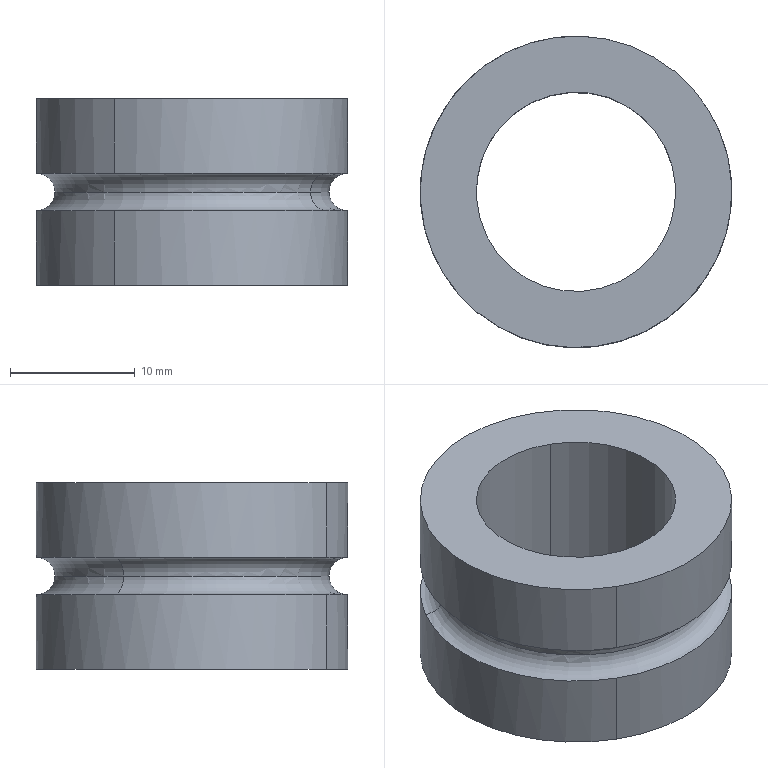Component | SolidWorks | SpindleFixtureAssemblyLeft-1_KLHFH016_16CopperSleeve-2 | 1 solid | 12 faces | box 25 x 25 x 15 mm | volume 4084 mm3 | cylinder 6 | torus 4 | plane 2 | commonest cylinder face diameters 25 x4 16 x2 | material Brass
build123d program:
from build123d import *

# Parameters (mm, degrees)
SKETCH1_R           = 12.5
SKETCH1_R_2         = 8
BOSS_EXTRUDE1_DEPTH = 7.5
SKETCH2_R           = 1.5


with BuildPart() as part:
    # Sketch1 → Boss-Extrude1 (new, symmetric)
    with BuildSketch(Plane.XY):
        Circle(SKETCH1_R)
        Circle(SKETCH1_R_2, mode=Mode.SUBTRACT)
    extrude(amount=BOSS_EXTRUDE1_DEPTH, both=True)

    # Sketch2 → Cut-Revolve1 (revolve, cut)
    with BuildSketch(Plane(origin=(0, 0, 0), x_dir=(0, 0, -1), z_dir=(1, 0, 0)), mode=Mode.PRIVATE) as cut_revolve1_sk:
        with Locations((0, 12.5)):
            Circle(SKETCH2_R)
    revolve(cut_revolve1_sk.sketch.rotate(Axis((0, 0, 0), (0, 0, -1)), 180), axis=Axis((0, 0, 0), (0, 0, -1)), mode=Mode.SUBTRACT)


solid = part.part

# Placed as in the assembly
solid = solid.moved(Location((-25, -43.301, -218.5), (0, 0, 0)))
STEP:
#1=CARTESIAN_POINT('',(-1.41,-1.459,-8.661));
#2=VERTEX_POINT('',#1);
#3=CARTESIAN_POINT('',(-1.359,-1.488,-8.602));
#4=VERTEX_POINT('',#3);
#5=CARTESIAN_POINT('',(-1.41,-1.459,-8.602));
#6=DIRECTION('',(-0.5,-0.866,0.));
#7=DIRECTION('',(0.866,-0.5,0.));
#8=AXIS2_PLACEMENT_3D('',#5,#6,#7);
#9=CIRCLE('',#8,0.05906);
#10=EDGE_CURVE('',#2,#4,#9,.T.);
#11=ORIENTED_EDGE('',*,*,#10,.T.);
#12=CARTESIAN_POINT('',(-0.6092,-1.921,-8.602));
#13=VERTEX_POINT('',#12);
#14=CARTESIAN_POINT('',(-0.9843,-1.705,-8.602));
#15=DIRECTION('',(0.,-0.,-1.));
#16=DIRECTION('',(-1.,0.,0.));
#17=AXIS2_PLACEMENT_3D('',#14,#15,#16);
#18=CIRCLE('',#17,0.4331);
#19=EDGE_CURVE('',#4,#13,#18,.T.);
#20=ORIENTED_EDGE('',*,*,#19,.T.);
#21=CARTESIAN_POINT('',(-0.5581,-1.951,-8.661));
#22=VERTEX_POINT('',#21);
#23=CARTESIAN_POINT('',(-0.5581,-1.951,-8.602));
#24=DIRECTION('',(0.5,0.866,-0.));
#25=DIRECTION('',(-0.866,0.5,0.));
#26=AXIS2_PLACEMENT_3D('',#23,#24,#25);
#27=CIRCLE('',#26,0.05906);
#28=EDGE_CURVE('',#22,#13,#27,.T.);
#29=ORIENTED_EDGE('',*,*,#28,.F.);
#30=CARTESIAN_POINT('',(-0.7382,-1.279,-8.661));
#31=VERTEX_POINT('',#30);
#32=CARTESIAN_POINT('',(-0.9843,-1.705,-8.661));
#33=DIRECTION('',(-0.,0.,1.));
#34=DIRECTION('',(0.866,-0.5,0.));
#35=AXIS2_PLACEMENT_3D('',#32,#33,#34);
#36=CIRCLE('',#35,0.4921);
#37=EDGE_CURVE('',#22,#31,#36,.T.);
#38=ORIENTED_EDGE('',*,*,#37,.T.);
#39=CARTESIAN_POINT('',(-0.9843,-1.705,-8.661));
#40=DIRECTION('',(-0.,0.,1.));
#41=DIRECTION('',(0.866,-0.5,0.));
#42=AXIS2_PLACEMENT_3D('',#39,#40,#41);
#43=CIRCLE('',#42,0.4921);
#44=EDGE_CURVE('',#31,#2,#43,.T.);
#45=ORIENTED_EDGE('',*,*,#44,.T.);
#46=EDGE_LOOP('',(#11,#20,#29,#38,#45));
#47=FACE_OUTER_BOUND('',#46,.T.);
#48=CARTESIAN_POINT('',(-0.9843,-1.705,-8.602));
#49=DIRECTION('',(0.,-0.,-1.));
#50=DIRECTION('',(-0.866,0.5,-0.));
#51=AXIS2_PLACEMENT_3D('',#48,#49,#50);
#52=TOROIDAL_SURFACE('',#51,0.4921,0.05906);
#53=ADVANCED_FACE('',(#47),#52,.F.);
#54=ORIENTED_EDGE('',*,*,#28,.T.);
#55=CARTESIAN_POINT('',(-0.9843,-1.705,-8.602));
#56=DIRECTION('',(0.,-0.,-1.));
#57=DIRECTION('',(-1.,0.,0.));
#58=AXIS2_PLACEMENT_3D('',#55,#56,#57);
#59=CIRCLE('',#58,0.4331);
#60=EDGE_CURVE('',#13,#4,#59,.T.);
#61=ORIENTED_EDGE('',*,*,#60,.T.);
#62=ORIENTED_EDGE('',*,*,#10,.F.);
#63=CARTESIAN_POINT('',(-1.23,-2.131,-8.661));
#64=VERTEX_POINT('',#63);
#65=CARTESIAN_POINT('',(-0.9843,-1.705,-8.661));
#66=DIRECTION('',(-0.,0.,1.));
#67=DIRECTION('',(0.866,-0.5,0.));
#68=AXIS2_PLACEMENT_3D('',#65,#66,#67);
#69=CIRCLE('',#68,0.4921);
#70=EDGE_CURVE('',#2,#64,#69,.T.);
#71=ORIENTED_EDGE('',*,*,#70,.T.);
#72=CARTESIAN_POINT('',(-0.9843,-1.705,-8.661));
#73=DIRECTION('',(-0.,0.,1.));
#74=DIRECTION('',(0.866,-0.5,0.));
#75=AXIS2_PLACEMENT_3D('',#72,#73,#74);
#76=CIRCLE('',#75,0.4921);
#77=EDGE_CURVE('',#64,#22,#76,.T.);
#78=ORIENTED_EDGE('',*,*,#77,.T.);
#79=EDGE_LOOP('',(#54,#61,#62,#71,#78));
#80=FACE_OUTER_BOUND('',#79,.T.);
#81=CARTESIAN_POINT('',(-0.9843,-1.705,-8.602));
#82=DIRECTION('',(0.,-0.,-1.));
#83=DIRECTION('',(-0.866,0.5,-0.));
#84=AXIS2_PLACEMENT_3D('',#81,#82,#83);
#85=TOROIDAL_SURFACE('',#84,0.4921,0.05906);
#86=ADVANCED_FACE('',(#80),#85,.F.);
#87=ORIENTED_EDGE('',*,*,#60,.F.);
#88=CARTESIAN_POINT('',(-0.5581,-1.951,-8.543));
#89=VERTEX_POINT('',#88);
#90=CARTESIAN_POINT('',(-0.5581,-1.951,-8.602));
#91=DIRECTION('',(0.5,0.866,-0.));
#92=DIRECTION('',(-0.866,0.5,0.));
#93=AXIS2_PLACEMENT_3D('',#90,#91,#92);
#94=CIRCLE('',#93,0.05906);
#95=EDGE_CURVE('',#13,#89,#94,.T.);
#96=ORIENTED_EDGE('',*,*,#95,.T.);
#97=CARTESIAN_POINT('',(-1.23,-2.131,-8.543));
#98=VERTEX_POINT('',#97);
#99=CARTESIAN_POINT('',(-0.9843,-1.705,-8.543));
#100=DIRECTION('',(0.,-0.,-1.));
#101=DIRECTION('',(-0.866,0.5,0.));
#102=AXIS2_PLACEMENT_3D('',#99,#100,#101);
#103=CIRCLE('',#102,0.4921);
#104=EDGE_CURVE('',#89,#98,#103,.T.);
#105=ORIENTED_EDGE('',*,*,#104,.T.);
#106=CARTESIAN_POINT('',(-1.41,-1.459,-8.543));
#107=VERTEX_POINT('',#106);
#108=CARTESIAN_POINT('',(-0.9843,-1.705,-8.543));
#109=DIRECTION('',(0.,-0.,-1.));
#110=DIRECTION('',(-0.866,0.5,0.));
#111=AXIS2_PLACEMENT_3D('',#108,#109,#110);
#112=CIRCLE('',#111,0.4921);
#113=EDGE_CURVE('',#98,#107,#112,.T.);
#114=ORIENTED_EDGE('',*,*,#113,.T.);
#115=CARTESIAN_POINT('',(-1.41,-1.459,-8.602));
#116=DIRECTION('',(-0.5,-0.866,0.));
#117=DIRECTION('',(0.866,-0.5,0.));
#118=AXIS2_PLACEMENT_3D('',#115,#116,#117);
#119=CIRCLE('',#118,0.05906);
#120=EDGE_CURVE('',#4,#107,#119,.T.);
#121=ORIENTED_EDGE('',*,*,#120,.F.);
#122=EDGE_LOOP('',(#87,#96,#105,#114,#121));
#123=FACE_OUTER_BOUND('',#122,.T.);
#124=CARTESIAN_POINT('',(-0.9843,-1.705,-8.602));
#125=DIRECTION('',(0.,-0.,-1.));
#126=DIRECTION('',(-0.866,0.5,-0.));
#127=AXIS2_PLACEMENT_3D('',#124,#125,#126);
#128=TOROIDAL_SURFACE('',#127,0.4921,0.05906);
#129=ADVANCED_FACE('',(#123),#128,.F.);
#130=CARTESIAN_POINT('',(-1.142,-1.978,-8.898));
#131=VERTEX_POINT('',#130);
#132=CARTESIAN_POINT('',(-0.8268,-1.432,-8.898));
#133=VERTEX_POINT('',#132);
#134=CARTESIAN_POINT('',(-0.9843,-1.705,-8.898));
#135=DIRECTION('',(0.,0.,-1.));
#136=DIRECTION('',(0.5,0.866,0.));
#137=AXIS2_PLACEMENT_3D('',#134,#135,#136);
#138=CIRCLE('',#137,0.315);
#139=EDGE_CURVE('',#131,#133,#138,.T.);
#140=ORIENTED_EDGE('',*,*,#139,.T.);
#141=CARTESIAN_POINT('',(-0.8268,-1.432,-8.307));
#142=VERTEX_POINT('',#141);
#143=CARTESIAN_POINT('',(-0.8268,-1.432,-8.898));
#144=DIRECTION('',(0.,0.,1.));
#145=VECTOR('',#144,39.37);
#146=LINE('',#143,#145);
#147=EDGE_CURVE('',#133,#142,#146,.T.);
#148=ORIENTED_EDGE('',*,*,#147,.T.);
#149=CARTESIAN_POINT('',(-1.142,-1.978,-8.307));
#150=VERTEX_POINT('',#149);
#151=CARTESIAN_POINT('',(-0.9843,-1.705,-8.307));
#152=DIRECTION('',(0.,0.,-1.));
#153=DIRECTION('',(0.5,0.866,0.));
#154=AXIS2_PLACEMENT_3D('',#151,#152,#153);
#155=CIRCLE('',#154,0.315);
#156=EDGE_CURVE('',#150,#142,#155,.T.);
#157=ORIENTED_EDGE('',*,*,#156,.F.);
#158=CARTESIAN_POINT('',(-1.142,-1.978,-8.898));
#159=DIRECTION('',(0.,0.,1.));
#160=VECTOR('',#159,39.37);
#161=LINE('',#158,#160);
#162=EDGE_CURVE('',#131,#150,#161,.T.);
#163=ORIENTED_EDGE('',*,*,#162,.F.);
#164=EDGE_LOOP('',(#140,#148,#157,#163));
#165=FACE_OUTER_BOUND('',#164,.T.);
#166=CARTESIAN_POINT('',(-0.9843,-1.705,-8.898));
#167=DIRECTION('',(0.,0.,1.));
#168=DIRECTION('',(-0.5,-0.866,0.));
#169=AXIS2_PLACEMENT_3D('',#166,#167,#168);
#170=CYLINDRICAL_SURFACE('',#169,0.315);
#171=ADVANCED_FACE('',(#165),#170,.F.);
#172=CARTESIAN_POINT('',(-0.7382,-1.279,-8.543));
#173=VERTEX_POINT('',#172);
#174=CARTESIAN_POINT('',(-0.9843,-1.705,-8.543));
#175=DIRECTION('',(0.,-0.,-1.));
#176=DIRECTION('',(-0.866,0.5,0.));
#177=AXIS2_PLACEMENT_3D('',#174,#175,#176);
#178=CIRCLE('',#177,0.4921);
#179=EDGE_CURVE('',#173,#89,#178,.T.);
#180=ORIENTED_EDGE('',*,*,#179,.F.);
#181=CARTESIAN_POINT('',(-0.7382,-1.279,-8.307));
#182=VERTEX_POINT('',#181);
#183=CARTESIAN_POINT('',(-0.7382,-1.279,-8.898));
#184=DIRECTION('',(0.,0.,1.));
#185=VECTOR('',#184,39.37);
#186=LINE('',#183,#185);
#187=EDGE_CURVE('',#173,#182,#186,.T.);
#188=ORIENTED_EDGE('',*,*,#187,.T.);
#189=CARTESIAN_POINT('',(-1.23,-2.131,-8.307));
#190=VERTEX_POINT('',#189);
#191=CARTESIAN_POINT('',(-0.9843,-1.705,-8.307));
#192=DIRECTION('',(0.,0.,-1.));
#193=DIRECTION('',(0.5,0.866,0.));
#194=AXIS2_PLACEMENT_3D('',#191,#192,#193);
#195=CIRCLE('',#194,0.4921);
#196=EDGE_CURVE('',#182,#190,#195,.T.);
#197=ORIENTED_EDGE('',*,*,#196,.T.);
#198=CARTESIAN_POINT('',(-1.23,-2.131,-8.898));
#199=DIRECTION('',(0.,0.,1.));
#200=VECTOR('',#199,39.37);
#201=LINE('',#198,#200);
#202=EDGE_CURVE('',#98,#190,#201,.T.);
#203=ORIENTED_EDGE('',*,*,#202,.F.);
#204=ORIENTED_EDGE('',*,*,#104,.F.);
#205=EDGE_LOOP('',(#180,#188,#197,#203,#204));
#206=FACE_OUTER_BOUND('',#205,.T.);
#207=CARTESIAN_POINT('',(-0.9843,-1.705,-8.898));
#208=DIRECTION('',(0.,0.,1.));
#209=DIRECTION('',(-0.5,-0.866,0.));
#210=AXIS2_PLACEMENT_3D('',#207,#208,#209);
#211=CYLINDRICAL_SURFACE('',#210,0.4921);
#212=ADVANCED_FACE('',(#206),#211,.T.);
#213=CARTESIAN_POINT('',(-0.7382,-1.279,-8.898));
#214=VERTEX_POINT('',#213);
#215=CARTESIAN_POINT('',(-1.23,-2.131,-8.898));
#216=VERTEX_POINT('',#215);
#217=CARTESIAN_POINT('',(-0.9843,-1.705,-8.898));
#218=DIRECTION('',(0.,0.,-1.));
#219=DIRECTION('',(0.5,0.866,0.));
#220=AXIS2_PLACEMENT_3D('',#217,#218,#219);
#221=CIRCLE('',#220,0.4921);
#222=EDGE_CURVE('',#214,#216,#221,.T.);
#223=ORIENTED_EDGE('',*,*,#222,.F.);
#224=CARTESIAN_POINT('',(-0.7382,-1.279,-8.898));
#225=DIRECTION('',(0.,0.,1.));
#226=VECTOR('',#225,39.37);
#227=LINE('',#224,#226);
#228=EDGE_CURVE('',#214,#31,#227,.T.);
#229=ORIENTED_EDGE('',*,*,#228,.T.);
#230=ORIENTED_EDGE('',*,*,#37,.F.);
#231=ORIENTED_EDGE('',*,*,#77,.F.);
#232=CARTESIAN_POINT('',(-1.23,-2.131,-8.898));
#233=DIRECTION('',(0.,0.,1.));
#234=VECTOR('',#233,39.37);
#235=LINE('',#232,#234);
#236=EDGE_CURVE('',#216,#64,#235,.T.);
#237=ORIENTED_EDGE('',*,*,#236,.F.);
#238=EDGE_LOOP('',(#223,#229,#230,#231,#237));
#239=FACE_OUTER_BOUND('',#238,.T.);
#240=CARTESIAN_POINT('',(-0.9843,-1.705,-8.898));
#241=DIRECTION('',(0.,0.,1.));
#242=DIRECTION('',(-0.5,-0.866,0.));
#243=AXIS2_PLACEMENT_3D('',#240,#241,#242);
#244=CYLINDRICAL_SURFACE('',#243,0.4921);
#245=ADVANCED_FACE('',(#239),#244,.T.);
#246=ORIENTED_EDGE('',*,*,#228,.F.);
#247=CARTESIAN_POINT('',(-0.9843,-1.705,-8.898));
#248=DIRECTION('',(0.,0.,-1.));
#249=DIRECTION('',(0.5,0.866,0.));
#250=AXIS2_PLACEMENT_3D('',#247,#248,#249);
#251=CIRCLE('',#250,0.4921);
#252=EDGE_CURVE('',#216,#214,#251,.T.);
#253=ORIENTED_EDGE('',*,*,#252,.F.);
#254=ORIENTED_EDGE('',*,*,#236,.T.);
#255=ORIENTED_EDGE('',*,*,#70,.F.);
#256=ORIENTED_EDGE('',*,*,#44,.F.);
#257=EDGE_LOOP('',(#246,#253,#254,#255,#256));
#258=FACE_OUTER_BOUND('',#257,.T.);
#259=CARTESIAN_POINT('',(-0.9843,-1.705,-8.898));
#260=DIRECTION('',(0.,0.,1.));
#261=DIRECTION('',(-0.5,-0.866,0.));
#262=AXIS2_PLACEMENT_3D('',#259,#260,#261);
#263=CYLINDRICAL_SURFACE('',#262,0.4921);
#264=ADVANCED_FACE('',(#258),#263,.T.);
#265=ORIENTED_EDGE('',*,*,#187,.F.);
#266=CARTESIAN_POINT('',(-0.9843,-1.705,-8.543));
#267=DIRECTION('',(0.,-0.,-1.));
#268=DIRECTION('',(-0.866,0.5,0.));
#269=AXIS2_PLACEMENT_3D('',#266,#267,#268);
#270=CIRCLE('',#269,0.4921);
#271=EDGE_CURVE('',#107,#173,#270,.T.);
#272=ORIENTED_EDGE('',*,*,#271,.F.);
#273=ORIENTED_EDGE('',*,*,#113,.F.);
#274=ORIENTED_EDGE('',*,*,#202,.T.);
#275=CARTESIAN_POINT('',(-0.9843,-1.705,-8.307));
#276=DIRECTION('',(0.,0.,-1.));
#277=DIRECTION('',(0.5,0.866,0.));
#278=AXIS2_PLACEMENT_3D('',#275,#276,#277);
#279=CIRCLE('',#278,0.4921);
#280=EDGE_CURVE('',#190,#182,#279,.T.);
#281=ORIENTED_EDGE('',*,*,#280,.T.);
#282=EDGE_LOOP('',(#265,#272,#273,#274,#281));
#283=FACE_OUTER_BOUND('',#282,.T.);
#284=CARTESIAN_POINT('',(-0.9843,-1.705,-8.898));
#285=DIRECTION('',(0.,0.,1.));
#286=DIRECTION('',(-0.5,-0.866,0.));
#287=AXIS2_PLACEMENT_3D('',#284,#285,#286);
#288=CYLINDRICAL_SURFACE('',#287,0.4921);
#289=ADVANCED_FACE('',(#283),#288,.T.);
#290=ORIENTED_EDGE('',*,*,#252,.T.);
#291=ORIENTED_EDGE('',*,*,#222,.T.);
#292=EDGE_LOOP('',(#290,#291));
#293=FACE_OUTER_BOUND('',#292,.T.);
#294=ORIENTED_EDGE('',*,*,#139,.F.);
#295=CARTESIAN_POINT('',(-0.9843,-1.705,-8.898));
#296=DIRECTION('',(0.,0.,-1.));
#297=DIRECTION('',(0.5,0.866,0.));
#298=AXIS2_PLACEMENT_3D('',#295,#296,#297);
#299=CIRCLE('',#298,0.315);
#300=EDGE_CURVE('',#133,#131,#299,.T.);
#301=ORIENTED_EDGE('',*,*,#300,.F.);
#302=EDGE_LOOP('',(#294,#301));
#303=FACE_BOUND('',#302,.T.);
#304=CARTESIAN_POINT('',(-0.9843,-1.705,-8.898));
#305=DIRECTION('',(0.,0.,-1.));
#306=DIRECTION('',(0.5,0.866,0.));
#307=AXIS2_PLACEMENT_3D('',#304,#305,#306);
#308=PLANE('',#307);
#309=ADVANCED_FACE('',(#293,#303),#308,.T.);
#310=ORIENTED_EDGE('',*,*,#280,.F.);
#311=ORIENTED_EDGE('',*,*,#196,.F.);
#312=EDGE_LOOP('',(#310,#311));
#313=FACE_OUTER_BOUND('',#312,.T.);
#314=ORIENTED_EDGE('',*,*,#156,.T.);
#315=CARTESIAN_POINT('',(-0.9843,-1.705,-8.307));
#316=DIRECTION('',(0.,0.,-1.));
#317=DIRECTION('',(0.5,0.866,0.));
#318=AXIS2_PLACEMENT_3D('',#315,#316,#317);
#319=CIRCLE('',#318,0.315);
#320=EDGE_CURVE('',#142,#150,#319,.T.);
#321=ORIENTED_EDGE('',*,*,#320,.T.);
#322=EDGE_LOOP('',(#314,#321));
#323=FACE_BOUND('',#322,.T.);
#324=CARTESIAN_POINT('',(-0.9843,-1.705,-8.307));
#325=DIRECTION('',(0.,0.,-1.));
#326=DIRECTION('',(0.5,0.866,0.));
#327=AXIS2_PLACEMENT_3D('',#324,#325,#326);
#328=PLANE('',#327);
#329=ADVANCED_FACE('',(#313,#323),#328,.F.);
#330=ORIENTED_EDGE('',*,*,#147,.F.);
#331=ORIENTED_EDGE('',*,*,#300,.T.);
#332=ORIENTED_EDGE('',*,*,#162,.T.);
#333=ORIENTED_EDGE('',*,*,#320,.F.);
#334=EDGE_LOOP('',(#330,#331,#332,#333));
#335=FACE_OUTER_BOUND('',#334,.T.);
#336=CARTESIAN_POINT('',(-0.9843,-1.705,-8.898));
#337=DIRECTION('',(0.,0.,1.));
#338=DIRECTION('',(-0.5,-0.866,0.));
#339=AXIS2_PLACEMENT_3D('',#336,#337,#338);
#340=CYLINDRICAL_SURFACE('',#339,0.315);
#341=ADVANCED_FACE('',(#335),#340,.F.);
#342=ORIENTED_EDGE('',*,*,#19,.F.);
#343=ORIENTED_EDGE('',*,*,#120,.T.);
#344=ORIENTED_EDGE('',*,*,#271,.T.);
#345=ORIENTED_EDGE('',*,*,#179,.T.);
#346=ORIENTED_EDGE('',*,*,#95,.F.);
#347=EDGE_LOOP('',(#342,#343,#344,#345,#346));
#348=FACE_OUTER_BOUND('',#347,.T.);
#349=CARTESIAN_POINT('',(-0.9843,-1.705,-8.602));
#350=DIRECTION('',(0.,-0.,-1.));
#351=DIRECTION('',(-0.866,0.5,-0.));
#352=AXIS2_PLACEMENT_3D('',#349,#350,#351);
#353=TOROIDAL_SURFACE('',#352,0.4921,0.05906);
#354=ADVANCED_FACE('',(#348),#353,.F.);
#355=CLOSED_SHELL('',(#53,#86,#129,#171,#212,#245,#264,#289,#309,#329,#341,#354));
#356=MANIFOLD_SOLID_BREP('',#355);
#357=CARTESIAN_POINT('',(0.,0.,0.));
#358=DIRECTION('',(0.,0.,1.));
#359=DIRECTION('',(1.,0.,0.));
#360=AXIS2_PLACEMENT_3D('',#357,#358,#359);
#361=(LENGTH_UNIT()NAMED_UNIT(*)SI_UNIT($,.METRE.));
#362=LENGTH_MEASURE_WITH_UNIT(LENGTH_MEASURE(0.0254),#361);
#363=DIMENSIONAL_EXPONENTS(1.,0.,0.,0.,0.,0.,0.);
#364=(CONVERSION_BASED_UNIT('',#362)LENGTH_UNIT()NAMED_UNIT(#363));
#365=UNCERTAINTY_MEASURE_WITH_UNIT(LENGTH_MEASURE(0.00001),#364,'','');
#366=(NAMED_UNIT(*)PLANE_ANGLE_UNIT()SI_UNIT($,.RADIAN.));
#367=(NAMED_UNIT(*)SI_UNIT($,.STERADIAN.)SOLID_ANGLE_UNIT());
#368=(GEOMETRIC_REPRESENTATION_CONTEXT(3)GLOBAL_UNCERTAINTY_ASSIGNED_CONTEXT((#365))GLOBAL_UNIT_ASSIGNED_CONTEXT((#364,#366,#367))REPRESENTATION_CONTEXT('',''));
#369=ADVANCED_BREP_SHAPE_REPRESENTATION('',(#356,#360),#368);
#370=COLOUR_RGB('',0.7922,0.8196,0.9333);
#371=FILL_AREA_STYLE_COLOUR('',#370);
#372=FILL_AREA_STYLE('',(#371));
#373=SURFACE_STYLE_FILL_AREA(#372);
#374=SURFACE_SIDE_STYLE('',(#373));
#375=SURFACE_STYLE_USAGE(.BOTH.,#374);
#376=PRESENTATION_STYLE_ASSIGNMENT((#375));
#377=STYLED_ITEM('',(#376),#356);
#378=PRESENTATION_LAYER_ASSIGNMENT('','',(#377));
#379=(LENGTH_UNIT()NAMED_UNIT(*)SI_UNIT($,.METRE.));
#380=LENGTH_MEASURE_WITH_UNIT(LENGTH_MEASURE(0.0254),#379);
#381=DIMENSIONAL_EXPONENTS(1.,0.,0.,0.,0.,0.,0.);
#382=(CONVERSION_BASED_UNIT('',#380)LENGTH_UNIT()NAMED_UNIT(#381));
#383=UNCERTAINTY_MEASURE_WITH_UNIT(LENGTH_MEASURE(0.00001),#382,'','');
#384=(NAMED_UNIT(*)PLANE_ANGLE_UNIT()SI_UNIT($,.RADIAN.));
#385=(NAMED_UNIT(*)SI_UNIT($,.STERADIAN.)SOLID_ANGLE_UNIT());
#386=(GEOMETRIC_REPRESENTATION_CONTEXT(3)GLOBAL_UNCERTAINTY_ASSIGNED_CONTEXT((#383))GLOBAL_UNIT_ASSIGNED_CONTEXT((#382,#384,#385))REPRESENTATION_CONTEXT('',''));
#387=MECHANICAL_DESIGN_GEOMETRIC_PRESENTATION_REPRESENTATION('',(#377),#386);